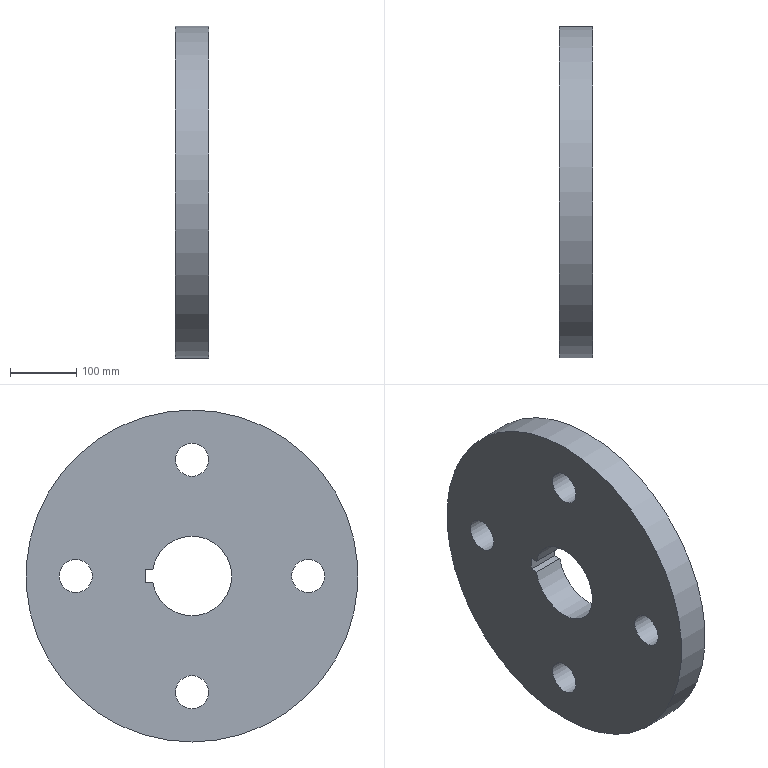Component | NX | ROTOR_DISC | 1 solid | 11 faces | box 50 x 500 x 500 mm | volume 8848841 mm3 | cylinder 6 | plane 5 | commonest cylinder face diameters 50 x4 500 x1 120 x1
STEP:
#1=CARTESIAN_POINT('',(0.,0.,0.));
#2=DIRECTION('',(0.,0.,1.));
#3=DIRECTION('',(1.,0.,0.));
#4=AXIS2_PLACEMENT_3D('',#1,#2,#3);
#5=CARTESIAN_POINT('',(641.458,-1109.721,829.997));
#6=VERTEX_POINT('',#5);
#7=CARTESIAN_POINT('',(641.458,-1098.711,829.997));
#8=VERTEX_POINT('',#7);
#9=CARTESIAN_POINT('',(641.458,-1109.721,829.997));
#10=DIRECTION('',(0.,1.,0.));
#11=VECTOR('',#10,1.);
#12=LINE('',#9,#11);
#13=CARTESIAN_POINT('',(591.458,-1109.721,829.997));
#14=DIRECTION('',(0.,0.,-1.));
#15=DIRECTION('',(-1.,0.,0.));
#16=AXIS2_PLACEMENT_3D('',#13,#14,#15);
#17=PLANE('',#16);
#18=CARTESIAN_POINT('',(-50.,0.));
#19=DIRECTION('',(0.,1.));
#20=VECTOR('',#19,1.);
#21=LINE('',#18,#20);
#22=(GEOMETRIC_REPRESENTATION_CONTEXT(2)PARAMETRIC_REPRESENTATION_CONTEXT()REPRESENTATION_CONTEXT('',''));
#23=DEFINITIONAL_REPRESENTATION('',(#21),#22);
#24=PCURVE('',#17,#23);
#25=CARTESIAN_POINT('',(641.458,-1168.882,839.997));
#26=DIRECTION('',(-1.,0.,0.));
#27=DIRECTION('',(0.,0.,1.));
#28=AXIS2_PLACEMENT_3D('',#25,#26,#27);
#29=PLANE('',#28);
#30=CARTESIAN_POINT('',(-10.,59.161));
#31=DIRECTION('',(0.,1.));
#32=VECTOR('',#31,1.);
#33=LINE('',#30,#32);
#34=(GEOMETRIC_REPRESENTATION_CONTEXT(2)PARAMETRIC_REPRESENTATION_CONTEXT()REPRESENTATION_CONTEXT('',''));
#35=DEFINITIONAL_REPRESENTATION('',(#33),#34);
#36=PCURVE('',#29,#35);
#37=SURFACE_CURVE('',#12,(#24,#36),.PCURVE_S1.);
#38=EDGE_CURVE('',#6,#8,#37,.T.);
#39=ORIENTED_EDGE('',*,*,#38,.T.);
#40=CARTESIAN_POINT('',(591.458,-1098.711,829.997));
#41=VERTEX_POINT('',#40);
#42=CARTESIAN_POINT('',(591.458,-1098.711,829.997));
#43=DIRECTION('',(1.,0.,0.));
#44=VECTOR('',#43,1.);
#45=LINE('',#42,#44);
#46=CARTESIAN_POINT('',(0.,11.01));
#47=DIRECTION('',(-1.,0.));
#48=VECTOR('',#47,1.);
#49=LINE('',#46,#48);
#50=(GEOMETRIC_REPRESENTATION_CONTEXT(2)PARAMETRIC_REPRESENTATION_CONTEXT()REPRESENTATION_CONTEXT('',''));
#51=DEFINITIONAL_REPRESENTATION('',(#49),#50);
#52=PCURVE('',#17,#51);
#53=CARTESIAN_POINT('',(591.458,-1098.711,829.997));
#54=DIRECTION('',(0.,1.,0.));
#55=DIRECTION('',(-1.,0.,0.));
#56=AXIS2_PLACEMENT_3D('',#53,#54,#55);
#57=PLANE('',#56);
#58=CARTESIAN_POINT('',(0.,0.));
#59=DIRECTION('',(-1.,0.));
#60=VECTOR('',#59,1.);
#61=LINE('',#58,#60);
#62=(GEOMETRIC_REPRESENTATION_CONTEXT(2)PARAMETRIC_REPRESENTATION_CONTEXT()REPRESENTATION_CONTEXT('',''));
#63=DEFINITIONAL_REPRESENTATION('',(#61),#62);
#64=PCURVE('',#57,#63);
#65=SURFACE_CURVE('',#45,(#52,#64),.PCURVE_S1.);
#66=EDGE_CURVE('',#41,#8,#65,.T.);
#67=ORIENTED_EDGE('',*,*,#66,.F.);
#68=CARTESIAN_POINT('',(591.458,-1109.721,829.997));
#69=VERTEX_POINT('',#68);
#70=CARTESIAN_POINT('',(591.458,-1109.721,829.997));
#71=DIRECTION('',(0.,1.,0.));
#72=VECTOR('',#71,1.);
#73=LINE('',#70,#72);
#74=CARTESIAN_POINT('',(0.,0.));
#75=DIRECTION('',(0.,1.));
#76=VECTOR('',#75,1.);
#77=LINE('',#74,#76);
#78=(GEOMETRIC_REPRESENTATION_CONTEXT(2)PARAMETRIC_REPRESENTATION_CONTEXT()REPRESENTATION_CONTEXT('',''));
#79=DEFINITIONAL_REPRESENTATION('',(#77),#78);
#80=PCURVE('',#17,#79);
#81=CARTESIAN_POINT('',(591.458,-1168.882,839.997));
#82=DIRECTION('',(-1.,0.,0.));
#83=DIRECTION('',(0.,0.,1.));
#84=AXIS2_PLACEMENT_3D('',#81,#82,#83);
#85=PLANE('',#84);
#86=CARTESIAN_POINT('',(-10.,59.161));
#87=DIRECTION('',(0.,1.));
#88=VECTOR('',#87,1.);
#89=LINE('',#86,#88);
#90=(GEOMETRIC_REPRESENTATION_CONTEXT(2)PARAMETRIC_REPRESENTATION_CONTEXT()REPRESENTATION_CONTEXT('',''));
#91=DEFINITIONAL_REPRESENTATION('',(#89),#90);
#92=PCURVE('',#85,#91);
#93=SURFACE_CURVE('',#73,(#80,#92),.PCURVE_S1.);
#94=EDGE_CURVE('',#69,#41,#93,.T.);
#95=ORIENTED_EDGE('',*,*,#94,.F.);
#96=CARTESIAN_POINT('',(591.458,-1109.721,829.997));
#97=DIRECTION('',(1.,0.,0.));
#98=VECTOR('',#97,1.);
#99=LINE('',#96,#98);
#100=CARTESIAN_POINT('',(0.,0.));
#101=DIRECTION('',(-1.,0.));
#102=VECTOR('',#101,1.);
#103=LINE('',#100,#102);
#104=(GEOMETRIC_REPRESENTATION_CONTEXT(2)PARAMETRIC_REPRESENTATION_CONTEXT()REPRESENTATION_CONTEXT('',''));
#105=DEFINITIONAL_REPRESENTATION('',(#103),#104);
#106=PCURVE('',#17,#105);
#107=CARTESIAN_POINT('',(591.458,-1168.882,839.997));
#108=DIRECTION('',(1.,0.,0.));
#109=DIRECTION('',(0.,0.,-1.));
#110=AXIS2_PLACEMENT_3D('',#107,#108,#109);
#111=CYLINDRICAL_SURFACE('',#110,60.);
#112=CARTESIAN_POINT('',(7.687,0.));
#113=DIRECTION('',(0.,1.));
#114=VECTOR('',#113,1.);
#115=LINE('',#112,#114);
#116=(GEOMETRIC_REPRESENTATION_CONTEXT(2)PARAMETRIC_REPRESENTATION_CONTEXT()REPRESENTATION_CONTEXT('',''));
#117=DEFINITIONAL_REPRESENTATION('',(#115),#116);
#118=PCURVE('',#111,#117);
#119=SURFACE_CURVE('',#99,(#106,#118),.PCURVE_S1.);
#120=EDGE_CURVE('',#69,#6,#119,.T.);
#121=ORIENTED_EDGE('',*,*,#120,.T.);
#122=EDGE_LOOP('',(#39,#67,#95,#121));
#123=FACE_BOUND('',#122,.T.);
#124=ADVANCED_FACE('',(#123),#17,.F.);
#125=CARTESIAN_POINT('',(641.458,-1098.711,849.997));
#126=VERTEX_POINT('',#125);
#127=CARTESIAN_POINT('',(641.458,-1098.711,829.997));
#128=DIRECTION('',(0.,0.,1.));
#129=VECTOR('',#128,1.);
#130=LINE('',#127,#129);
#131=CARTESIAN_POINT('',(-50.,0.));
#132=DIRECTION('',(0.,1.));
#133=VECTOR('',#132,1.);
#134=LINE('',#131,#133);
#135=(GEOMETRIC_REPRESENTATION_CONTEXT(2)PARAMETRIC_REPRESENTATION_CONTEXT()REPRESENTATION_CONTEXT('',''));
#136=DEFINITIONAL_REPRESENTATION('',(#134),#135);
#137=PCURVE('',#57,#136);
#138=CARTESIAN_POINT('',(-10.,70.171));
#139=DIRECTION('',(1.,0.));
#140=VECTOR('',#139,1.);
#141=LINE('',#138,#140);
#142=(GEOMETRIC_REPRESENTATION_CONTEXT(2)PARAMETRIC_REPRESENTATION_CONTEXT()REPRESENTATION_CONTEXT('',''));
#143=DEFINITIONAL_REPRESENTATION('',(#141),#142);
#144=PCURVE('',#29,#143);
#145=SURFACE_CURVE('',#130,(#137,#144),.PCURVE_S1.);
#146=EDGE_CURVE('',#8,#126,#145,.T.);
#147=ORIENTED_EDGE('',*,*,#146,.T.);
#148=CARTESIAN_POINT('',(591.458,-1098.711,849.997));
#149=VERTEX_POINT('',#148);
#150=CARTESIAN_POINT('',(591.458,-1098.711,849.997));
#151=DIRECTION('',(1.,0.,0.));
#152=VECTOR('',#151,1.);
#153=LINE('',#150,#152);
#154=CARTESIAN_POINT('',(0.,20.));
#155=DIRECTION('',(-1.,0.));
#156=VECTOR('',#155,1.);
#157=LINE('',#154,#156);
#158=(GEOMETRIC_REPRESENTATION_CONTEXT(2)PARAMETRIC_REPRESENTATION_CONTEXT()REPRESENTATION_CONTEXT('',''));
#159=DEFINITIONAL_REPRESENTATION('',(#157),#158);
#160=PCURVE('',#57,#159);
#161=CARTESIAN_POINT('',(591.458,-1098.711,849.997));
#162=DIRECTION('',(0.,0.,1.));
#163=DIRECTION('',(1.,0.,0.));
#164=AXIS2_PLACEMENT_3D('',#161,#162,#163);
#165=PLANE('',#164);
#166=CARTESIAN_POINT('',(0.,0.));
#167=DIRECTION('',(1.,0.));
#168=VECTOR('',#167,1.);
#169=LINE('',#166,#168);
#170=(GEOMETRIC_REPRESENTATION_CONTEXT(2)PARAMETRIC_REPRESENTATION_CONTEXT()REPRESENTATION_CONTEXT('',''));
#171=DEFINITIONAL_REPRESENTATION('',(#169),#170);
#172=PCURVE('',#165,#171);
#173=SURFACE_CURVE('',#153,(#160,#172),.PCURVE_S1.);
#174=EDGE_CURVE('',#149,#126,#173,.T.);
#175=ORIENTED_EDGE('',*,*,#174,.F.);
#176=CARTESIAN_POINT('',(591.458,-1098.711,829.997));
#177=DIRECTION('',(0.,0.,1.));
#178=VECTOR('',#177,1.);
#179=LINE('',#176,#178);
#180=CARTESIAN_POINT('',(0.,0.));
#181=DIRECTION('',(0.,1.));
#182=VECTOR('',#181,1.);
#183=LINE('',#180,#182);
#184=(GEOMETRIC_REPRESENTATION_CONTEXT(2)PARAMETRIC_REPRESENTATION_CONTEXT()REPRESENTATION_CONTEXT('',''));
#185=DEFINITIONAL_REPRESENTATION('',(#183),#184);
#186=PCURVE('',#57,#185);
#187=CARTESIAN_POINT('',(-10.,70.171));
#188=DIRECTION('',(1.,0.));
#189=VECTOR('',#188,1.);
#190=LINE('',#187,#189);
#191=(GEOMETRIC_REPRESENTATION_CONTEXT(2)PARAMETRIC_REPRESENTATION_CONTEXT()REPRESENTATION_CONTEXT('',''));
#192=DEFINITIONAL_REPRESENTATION('',(#190),#191);
#193=PCURVE('',#85,#192);
#194=SURFACE_CURVE('',#179,(#186,#193),.PCURVE_S1.);
#195=EDGE_CURVE('',#41,#149,#194,.T.);
#196=ORIENTED_EDGE('',*,*,#195,.F.);
#197=ORIENTED_EDGE('',*,*,#66,.T.);
#198=EDGE_LOOP('',(#147,#175,#196,#197));
#199=FACE_BOUND('',#198,.T.);
#200=ADVANCED_FACE('',(#199),#57,.F.);
#201=CARTESIAN_POINT('',(641.458,-1109.721,849.997));
#202=VERTEX_POINT('',#201);
#203=CARTESIAN_POINT('',(641.458,-1098.711,849.997));
#204=DIRECTION('',(0.,-1.,0.));
#205=VECTOR('',#204,1.);
#206=LINE('',#203,#205);
#207=CARTESIAN_POINT('',(50.,0.));
#208=DIRECTION('',(0.,-1.));
#209=VECTOR('',#208,1.);
#210=LINE('',#207,#209);
#211=(GEOMETRIC_REPRESENTATION_CONTEXT(2)PARAMETRIC_REPRESENTATION_CONTEXT()REPRESENTATION_CONTEXT('',''));
#212=DEFINITIONAL_REPRESENTATION('',(#210),#211);
#213=PCURVE('',#165,#212);
#214=CARTESIAN_POINT('',(10.,70.171));
#215=DIRECTION('',(0.,-1.));
#216=VECTOR('',#215,1.);
#217=LINE('',#214,#216);
#218=(GEOMETRIC_REPRESENTATION_CONTEXT(2)PARAMETRIC_REPRESENTATION_CONTEXT()REPRESENTATION_CONTEXT('',''));
#219=DEFINITIONAL_REPRESENTATION('',(#217),#218);
#220=PCURVE('',#29,#219);
#221=SURFACE_CURVE('',#206,(#213,#220),.PCURVE_S1.);
#222=EDGE_CURVE('',#126,#202,#221,.T.);
#223=ORIENTED_EDGE('',*,*,#222,.T.);
#224=CARTESIAN_POINT('',(591.458,-1109.721,849.997));
#225=VERTEX_POINT('',#224);
#226=CARTESIAN_POINT('',(591.458,-1109.721,849.997));
#227=DIRECTION('',(1.,0.,0.));
#228=VECTOR('',#227,1.);
#229=LINE('',#226,#228);
#230=CARTESIAN_POINT('',(0.,-11.01));
#231=DIRECTION('',(1.,0.));
#232=VECTOR('',#231,1.);
#233=LINE('',#230,#232);
#234=(GEOMETRIC_REPRESENTATION_CONTEXT(2)PARAMETRIC_REPRESENTATION_CONTEXT()REPRESENTATION_CONTEXT('',''));
#235=DEFINITIONAL_REPRESENTATION('',(#233),#234);
#236=PCURVE('',#165,#235);
#237=CARTESIAN_POINT('',(1.738,0.));
#238=DIRECTION('',(0.,1.));
#239=VECTOR('',#238,1.);
#240=LINE('',#237,#239);
#241=(GEOMETRIC_REPRESENTATION_CONTEXT(2)PARAMETRIC_REPRESENTATION_CONTEXT()REPRESENTATION_CONTEXT('',''));
#242=DEFINITIONAL_REPRESENTATION('',(#240),#241);
#243=PCURVE('',#111,#242);
#244=SURFACE_CURVE('',#229,(#236,#243),.PCURVE_S1.);
#245=EDGE_CURVE('',#225,#202,#244,.T.);
#246=ORIENTED_EDGE('',*,*,#245,.F.);
#247=CARTESIAN_POINT('',(591.458,-1098.711,849.997));
#248=DIRECTION('',(0.,-1.,0.));
#249=VECTOR('',#248,1.);
#250=LINE('',#247,#249);
#251=CARTESIAN_POINT('',(0.,0.));
#252=DIRECTION('',(0.,-1.));
#253=VECTOR('',#252,1.);
#254=LINE('',#251,#253);
#255=(GEOMETRIC_REPRESENTATION_CONTEXT(2)PARAMETRIC_REPRESENTATION_CONTEXT()REPRESENTATION_CONTEXT('',''));
#256=DEFINITIONAL_REPRESENTATION('',(#254),#255);
#257=PCURVE('',#165,#256);
#258=CARTESIAN_POINT('',(10.,70.171));
#259=DIRECTION('',(0.,-1.));
#260=VECTOR('',#259,1.);
#261=LINE('',#258,#260);
#262=(GEOMETRIC_REPRESENTATION_CONTEXT(2)PARAMETRIC_REPRESENTATION_CONTEXT()REPRESENTATION_CONTEXT('',''));
#263=DEFINITIONAL_REPRESENTATION('',(#261),#262);
#264=PCURVE('',#85,#263);
#265=SURFACE_CURVE('',#250,(#257,#264),.PCURVE_S1.);
#266=EDGE_CURVE('',#149,#225,#265,.T.);
#267=ORIENTED_EDGE('',*,*,#266,.F.);
#268=ORIENTED_EDGE('',*,*,#174,.T.);
#269=EDGE_LOOP('',(#223,#246,#267,#268));
#270=FACE_BOUND('',#269,.T.);
#271=ADVANCED_FACE('',(#270),#165,.F.);
#272=CARTESIAN_POINT('',(591.458,-1168.882,639.997));
#273=VERTEX_POINT('',#272);
#274=CARTESIAN_POINT('',(591.458,-1168.882,664.997));
#275=DIRECTION('',(-1.,0.,0.));
#276=DIRECTION('',(0.,0.,-1.));
#277=AXIS2_PLACEMENT_3D('',#274,#275,#276);
#278=CIRCLE('',#277,25.);
#279=CARTESIAN_POINT('',(591.458,-1168.882,664.997));
#280=DIRECTION('',(1.,0.,0.));
#281=DIRECTION('',(0.,0.,-1.));
#282=AXIS2_PLACEMENT_3D('',#279,#280,#281);
#283=CYLINDRICAL_SURFACE('',#282,25.);
#284=CARTESIAN_POINT('',(6.283,0.));
#285=DIRECTION('',(-1.,0.));
#286=VECTOR('',#285,1.);
#287=LINE('',#284,#286);
#288=(GEOMETRIC_REPRESENTATION_CONTEXT(2)PARAMETRIC_REPRESENTATION_CONTEXT()REPRESENTATION_CONTEXT('',''));
#289=DEFINITIONAL_REPRESENTATION('',(#287),#288);
#290=PCURVE('',#283,#289);
#291=CARTESIAN_POINT('',(-175.,0.));
#292=DIRECTION('',(-1.,0.));
#293=AXIS2_PLACEMENT_2D('',#291,#292);
#294=CIRCLE('',#293,25.);
#295=(GEOMETRIC_REPRESENTATION_CONTEXT(2)PARAMETRIC_REPRESENTATION_CONTEXT()REPRESENTATION_CONTEXT('',''));
#296=DEFINITIONAL_REPRESENTATION('',(#294),#295);
#297=PCURVE('',#85,#296);
#298=SURFACE_CURVE('',#278,(#290,#297),.PCURVE_S1.);
#299=EDGE_CURVE('',#273,#273,#298,.T.);
#300=ORIENTED_EDGE('',*,*,#299,.F.);
#301=CARTESIAN_POINT('',(641.458,-1168.882,639.997));
#302=VERTEX_POINT('',#301);
#303=CARTESIAN_POINT('',(591.458,-1168.882,639.997));
#304=CARTESIAN_POINT('',(641.458,-1168.882,639.997));
#305=B_SPLINE_CURVE_WITH_KNOTS('',1,(#303,#304),.UNSPECIFIED.,.F.,.F.,(2,2),(0.,50.),.PIECEWISE_BEZIER_KNOTS.);
#306=CARTESIAN_POINT('',(6.283,0.));
#307=DIRECTION('',(0.,1.));
#308=VECTOR('',#307,1.);
#309=LINE('',#306,#308);
#310=(GEOMETRIC_REPRESENTATION_CONTEXT(2)PARAMETRIC_REPRESENTATION_CONTEXT()REPRESENTATION_CONTEXT('',''));
#311=DEFINITIONAL_REPRESENTATION('',(#309),#310);
#312=PCURVE('',#283,#311);
#313=CARTESIAN_POINT('',(0.,0.));
#314=DIRECTION('',(0.,1.));
#315=VECTOR('',#314,1.);
#316=LINE('',#313,#315);
#317=(GEOMETRIC_REPRESENTATION_CONTEXT(2)PARAMETRIC_REPRESENTATION_CONTEXT()REPRESENTATION_CONTEXT('',''));
#318=DEFINITIONAL_REPRESENTATION('',(#316),#317);
#319=PCURVE('',#283,#318);
#320=SEAM_CURVE('',#305,(#312,#319),.PCURVE_S1.);
#321=EDGE_CURVE('',#273,#302,#320,.T.);
#322=ORIENTED_EDGE('',*,*,#321,.T.);
#323=CARTESIAN_POINT('',(641.458,-1168.882,664.997));
#324=DIRECTION('',(-1.,0.,0.));
#325=DIRECTION('',(0.,0.,-1.));
#326=AXIS2_PLACEMENT_3D('',#323,#324,#325);
#327=CIRCLE('',#326,25.);
#328=CARTESIAN_POINT('',(6.283,50.));
#329=DIRECTION('',(-1.,0.));
#330=VECTOR('',#329,1.);
#331=LINE('',#328,#330);
#332=(GEOMETRIC_REPRESENTATION_CONTEXT(2)PARAMETRIC_REPRESENTATION_CONTEXT()REPRESENTATION_CONTEXT('',''));
#333=DEFINITIONAL_REPRESENTATION('',(#331),#332);
#334=PCURVE('',#283,#333);
#335=CARTESIAN_POINT('',(-175.,0.));
#336=DIRECTION('',(-1.,0.));
#337=AXIS2_PLACEMENT_2D('',#335,#336);
#338=CIRCLE('',#337,25.);
#339=(GEOMETRIC_REPRESENTATION_CONTEXT(2)PARAMETRIC_REPRESENTATION_CONTEXT()REPRESENTATION_CONTEXT('',''));
#340=DEFINITIONAL_REPRESENTATION('',(#338),#339);
#341=PCURVE('',#29,#340);
#342=SURFACE_CURVE('',#327,(#334,#341),.PCURVE_S1.);
#343=EDGE_CURVE('',#302,#302,#342,.T.);
#344=ORIENTED_EDGE('',*,*,#343,.T.);
#345=ORIENTED_EDGE('',*,*,#321,.F.);
#346=EDGE_LOOP('',(#300,#322,#344,#345));
#347=FACE_BOUND('',#346,.F.);
#348=ADVANCED_FACE('',(#347),#283,.F.);
#349=CARTESIAN_POINT('',(591.458,-1368.882,839.997));
#350=VERTEX_POINT('',#349);
#351=CARTESIAN_POINT('',(591.458,-1343.882,839.997));
#352=DIRECTION('',(-1.,0.,0.));
#353=DIRECTION('',(0.,-1.,0.));
#354=AXIS2_PLACEMENT_3D('',#351,#352,#353);
#355=CIRCLE('',#354,25.);
#356=CARTESIAN_POINT('',(591.458,-1343.882,839.997));
#357=DIRECTION('',(1.,0.,0.));
#358=DIRECTION('',(0.,0.,-1.));
#359=AXIS2_PLACEMENT_3D('',#356,#357,#358);
#360=CYLINDRICAL_SURFACE('',#359,25.);
#361=CARTESIAN_POINT('',(10.996,0.));
#362=DIRECTION('',(-1.,0.));
#363=VECTOR('',#362,1.);
#364=LINE('',#361,#363);
#365=(GEOMETRIC_REPRESENTATION_CONTEXT(2)PARAMETRIC_REPRESENTATION_CONTEXT()REPRESENTATION_CONTEXT('',''));
#366=DEFINITIONAL_REPRESENTATION('',(#364),#365);
#367=PCURVE('',#360,#366);
#368=CARTESIAN_POINT('',(0.,-175.));
#369=DIRECTION('',(0.,-1.));
#370=AXIS2_PLACEMENT_2D('',#368,#369);
#371=CIRCLE('',#370,25.);
#372=(GEOMETRIC_REPRESENTATION_CONTEXT(2)PARAMETRIC_REPRESENTATION_CONTEXT()REPRESENTATION_CONTEXT('',''));
#373=DEFINITIONAL_REPRESENTATION('',(#371),#372);
#374=PCURVE('',#85,#373);
#375=SURFACE_CURVE('',#355,(#367,#374),.PCURVE_S1.);
#376=EDGE_CURVE('',#350,#350,#375,.T.);
#377=ORIENTED_EDGE('',*,*,#376,.F.);
#378=CARTESIAN_POINT('',(641.458,-1368.882,839.997));
#379=VERTEX_POINT('',#378);
#380=CARTESIAN_POINT('',(591.458,-1368.882,839.997));
#381=CARTESIAN_POINT('',(641.458,-1368.882,839.997));
#382=B_SPLINE_CURVE_WITH_KNOTS('',1,(#380,#381),.UNSPECIFIED.,.F.,.F.,(2,2),(0.,50.),.PIECEWISE_BEZIER_KNOTS.);
#383=CARTESIAN_POINT('',(10.996,0.));
#384=DIRECTION('',(0.,1.));
#385=VECTOR('',#384,1.);
#386=LINE('',#383,#385);
#387=(GEOMETRIC_REPRESENTATION_CONTEXT(2)PARAMETRIC_REPRESENTATION_CONTEXT()REPRESENTATION_CONTEXT('',''));
#388=DEFINITIONAL_REPRESENTATION('',(#386),#387);
#389=PCURVE('',#360,#388);
#390=CARTESIAN_POINT('',(4.712,0.));
#391=DIRECTION('',(0.,1.));
#392=VECTOR('',#391,1.);
#393=LINE('',#390,#392);
#394=(GEOMETRIC_REPRESENTATION_CONTEXT(2)PARAMETRIC_REPRESENTATION_CONTEXT()REPRESENTATION_CONTEXT('',''));
#395=DEFINITIONAL_REPRESENTATION('',(#393),#394);
#396=PCURVE('',#360,#395);
#397=SEAM_CURVE('',#382,(#389,#396),.PCURVE_S1.);
#398=EDGE_CURVE('',#350,#379,#397,.T.);
#399=ORIENTED_EDGE('',*,*,#398,.T.);
#400=CARTESIAN_POINT('',(641.458,-1343.882,839.997));
#401=DIRECTION('',(-1.,0.,0.));
#402=DIRECTION('',(0.,-1.,0.));
#403=AXIS2_PLACEMENT_3D('',#400,#401,#402);
#404=CIRCLE('',#403,25.);
#405=CARTESIAN_POINT('',(10.996,50.));
#406=DIRECTION('',(-1.,0.));
#407=VECTOR('',#406,1.);
#408=LINE('',#405,#407);
#409=(GEOMETRIC_REPRESENTATION_CONTEXT(2)PARAMETRIC_REPRESENTATION_CONTEXT()REPRESENTATION_CONTEXT('',''));
#410=DEFINITIONAL_REPRESENTATION('',(#408),#409);
#411=PCURVE('',#360,#410);
#412=CARTESIAN_POINT('',(0.,-175.));
#413=DIRECTION('',(0.,-1.));
#414=AXIS2_PLACEMENT_2D('',#412,#413);
#415=CIRCLE('',#414,25.);
#416=(GEOMETRIC_REPRESENTATION_CONTEXT(2)PARAMETRIC_REPRESENTATION_CONTEXT()REPRESENTATION_CONTEXT('',''));
#417=DEFINITIONAL_REPRESENTATION('',(#415),#416);
#418=PCURVE('',#29,#417);
#419=SURFACE_CURVE('',#404,(#411,#418),.PCURVE_S1.);
#420=EDGE_CURVE('',#379,#379,#419,.T.);
#421=ORIENTED_EDGE('',*,*,#420,.T.);
#422=ORIENTED_EDGE('',*,*,#398,.F.);
#423=EDGE_LOOP('',(#377,#399,#421,#422));
#424=FACE_BOUND('',#423,.F.);
#425=ADVANCED_FACE('',(#424),#360,.F.);
#426=CARTESIAN_POINT('',(591.458,-968.882,839.997));
#427=VERTEX_POINT('',#426);
#428=CARTESIAN_POINT('',(591.458,-993.882,839.997));
#429=DIRECTION('',(-1.,0.,0.));
#430=DIRECTION('',(0.,1.,0.));
#431=AXIS2_PLACEMENT_3D('',#428,#429,#430);
#432=CIRCLE('',#431,25.);
#433=CARTESIAN_POINT('',(591.458,-993.882,839.997));
#434=DIRECTION('',(1.,0.,0.));
#435=DIRECTION('',(0.,0.,-1.));
#436=AXIS2_PLACEMENT_3D('',#433,#434,#435);
#437=CYLINDRICAL_SURFACE('',#436,25.);
#438=CARTESIAN_POINT('',(7.854,0.));
#439=DIRECTION('',(-1.,0.));
#440=VECTOR('',#439,1.);
#441=LINE('',#438,#440);
#442=(GEOMETRIC_REPRESENTATION_CONTEXT(2)PARAMETRIC_REPRESENTATION_CONTEXT()REPRESENTATION_CONTEXT('',''));
#443=DEFINITIONAL_REPRESENTATION('',(#441),#442);
#444=PCURVE('',#437,#443);
#445=CARTESIAN_POINT('',(0.,175.));
#446=DIRECTION('',(0.,1.));
#447=AXIS2_PLACEMENT_2D('',#445,#446);
#448=CIRCLE('',#447,25.);
#449=(GEOMETRIC_REPRESENTATION_CONTEXT(2)PARAMETRIC_REPRESENTATION_CONTEXT()REPRESENTATION_CONTEXT('',''));
#450=DEFINITIONAL_REPRESENTATION('',(#448),#449);
#451=PCURVE('',#85,#450);
#452=SURFACE_CURVE('',#432,(#444,#451),.PCURVE_S1.);
#453=EDGE_CURVE('',#427,#427,#452,.T.);
#454=ORIENTED_EDGE('',*,*,#453,.F.);
#455=CARTESIAN_POINT('',(641.458,-968.882,839.997));
#456=VERTEX_POINT('',#455);
#457=CARTESIAN_POINT('',(591.458,-968.882,839.997));
#458=CARTESIAN_POINT('',(641.458,-968.882,839.997));
#459=B_SPLINE_CURVE_WITH_KNOTS('',1,(#457,#458),.UNSPECIFIED.,.F.,.F.,(2,2),(0.,50.),.PIECEWISE_BEZIER_KNOTS.);
#460=CARTESIAN_POINT('',(7.854,0.));
#461=DIRECTION('',(0.,1.));
#462=VECTOR('',#461,1.);
#463=LINE('',#460,#462);
#464=(GEOMETRIC_REPRESENTATION_CONTEXT(2)PARAMETRIC_REPRESENTATION_CONTEXT()REPRESENTATION_CONTEXT('',''));
#465=DEFINITIONAL_REPRESENTATION('',(#463),#464);
#466=PCURVE('',#437,#465);
#467=CARTESIAN_POINT('',(1.571,0.));
#468=DIRECTION('',(0.,1.));
#469=VECTOR('',#468,1.);
#470=LINE('',#467,#469);
#471=(GEOMETRIC_REPRESENTATION_CONTEXT(2)PARAMETRIC_REPRESENTATION_CONTEXT()REPRESENTATION_CONTEXT('',''));
#472=DEFINITIONAL_REPRESENTATION('',(#470),#471);
#473=PCURVE('',#437,#472);
#474=SEAM_CURVE('',#459,(#466,#473),.PCURVE_S1.);
#475=EDGE_CURVE('',#427,#456,#474,.T.);
#476=ORIENTED_EDGE('',*,*,#475,.T.);
#477=CARTESIAN_POINT('',(641.458,-993.882,839.997));
#478=DIRECTION('',(-1.,0.,0.));
#479=DIRECTION('',(0.,1.,0.));
#480=AXIS2_PLACEMENT_3D('',#477,#478,#479);
#481=CIRCLE('',#480,25.);
#482=CARTESIAN_POINT('',(7.854,50.));
#483=DIRECTION('',(-1.,0.));
#484=VECTOR('',#483,1.);
#485=LINE('',#482,#484);
#486=(GEOMETRIC_REPRESENTATION_CONTEXT(2)PARAMETRIC_REPRESENTATION_CONTEXT()REPRESENTATION_CONTEXT('',''));
#487=DEFINITIONAL_REPRESENTATION('',(#485),#486);
#488=PCURVE('',#437,#487);
#489=CARTESIAN_POINT('',(0.,175.));
#490=DIRECTION('',(0.,1.));
#491=AXIS2_PLACEMENT_2D('',#489,#490);
#492=CIRCLE('',#491,25.);
#493=(GEOMETRIC_REPRESENTATION_CONTEXT(2)PARAMETRIC_REPRESENTATION_CONTEXT()REPRESENTATION_CONTEXT('',''));
#494=DEFINITIONAL_REPRESENTATION('',(#492),#493);
#495=PCURVE('',#29,#494);
#496=SURFACE_CURVE('',#481,(#488,#495),.PCURVE_S1.);
#497=EDGE_CURVE('',#456,#456,#496,.T.);
#498=ORIENTED_EDGE('',*,*,#497,.T.);
#499=ORIENTED_EDGE('',*,*,#475,.F.);
#500=EDGE_LOOP('',(#454,#476,#498,#499));
#501=FACE_BOUND('',#500,.F.);
#502=ADVANCED_FACE('',(#501),#437,.F.);
#503=CARTESIAN_POINT('',(591.458,-1168.882,1039.997));
#504=VERTEX_POINT('',#503);
#505=CARTESIAN_POINT('',(591.458,-1168.882,1014.997));
#506=DIRECTION('',(-1.,0.,0.));
#507=DIRECTION('',(0.,0.,1.));
#508=AXIS2_PLACEMENT_3D('',#505,#506,#507);
#509=CIRCLE('',#508,25.);
#510=CARTESIAN_POINT('',(591.458,-1168.882,1014.997));
#511=DIRECTION('',(1.,0.,0.));
#512=DIRECTION('',(0.,0.,-1.));
#513=AXIS2_PLACEMENT_3D('',#510,#511,#512);
#514=CYLINDRICAL_SURFACE('',#513,25.);
#515=CARTESIAN_POINT('',(9.425,0.));
#516=DIRECTION('',(-1.,0.));
#517=VECTOR('',#516,1.);
#518=LINE('',#515,#517);
#519=(GEOMETRIC_REPRESENTATION_CONTEXT(2)PARAMETRIC_REPRESENTATION_CONTEXT()REPRESENTATION_CONTEXT('',''));
#520=DEFINITIONAL_REPRESENTATION('',(#518),#519);
#521=PCURVE('',#514,#520);
#522=CARTESIAN_POINT('',(175.,0.));
#523=DIRECTION('',(1.,0.));
#524=AXIS2_PLACEMENT_2D('',#522,#523);
#525=CIRCLE('',#524,25.);
#526=(GEOMETRIC_REPRESENTATION_CONTEXT(2)PARAMETRIC_REPRESENTATION_CONTEXT()REPRESENTATION_CONTEXT('',''));
#527=DEFINITIONAL_REPRESENTATION('',(#525),#526);
#528=PCURVE('',#85,#527);
#529=SURFACE_CURVE('',#509,(#521,#528),.PCURVE_S1.);
#530=EDGE_CURVE('',#504,#504,#529,.T.);
#531=ORIENTED_EDGE('',*,*,#530,.F.);
#532=CARTESIAN_POINT('',(641.458,-1168.882,1039.997));
#533=VERTEX_POINT('',#532);
#534=CARTESIAN_POINT('',(591.458,-1168.882,1039.997));
#535=CARTESIAN_POINT('',(641.458,-1168.882,1039.997));
#536=B_SPLINE_CURVE_WITH_KNOTS('',1,(#534,#535),.UNSPECIFIED.,.F.,.F.,(2,2),(0.,50.),.PIECEWISE_BEZIER_KNOTS.);
#537=CARTESIAN_POINT('',(9.425,0.));
#538=DIRECTION('',(0.,1.));
#539=VECTOR('',#538,1.);
#540=LINE('',#537,#539);
#541=(GEOMETRIC_REPRESENTATION_CONTEXT(2)PARAMETRIC_REPRESENTATION_CONTEXT()REPRESENTATION_CONTEXT('',''));
#542=DEFINITIONAL_REPRESENTATION('',(#540),#541);
#543=PCURVE('',#514,#542);
#544=CARTESIAN_POINT('',(3.142,0.));
#545=DIRECTION('',(0.,1.));
#546=VECTOR('',#545,1.);
#547=LINE('',#544,#546);
#548=(GEOMETRIC_REPRESENTATION_CONTEXT(2)PARAMETRIC_REPRESENTATION_CONTEXT()REPRESENTATION_CONTEXT('',''));
#549=DEFINITIONAL_REPRESENTATION('',(#547),#548);
#550=PCURVE('',#514,#549);
#551=SEAM_CURVE('',#536,(#543,#550),.PCURVE_S1.);
#552=EDGE_CURVE('',#504,#533,#551,.T.);
#553=ORIENTED_EDGE('',*,*,#552,.T.);
#554=CARTESIAN_POINT('',(641.458,-1168.882,1014.997));
#555=DIRECTION('',(-1.,0.,0.));
#556=DIRECTION('',(0.,0.,1.));
#557=AXIS2_PLACEMENT_3D('',#554,#555,#556);
#558=CIRCLE('',#557,25.);
#559=CARTESIAN_POINT('',(9.425,50.));
#560=DIRECTION('',(-1.,0.));
#561=VECTOR('',#560,1.);
#562=LINE('',#559,#561);
#563=(GEOMETRIC_REPRESENTATION_CONTEXT(2)PARAMETRIC_REPRESENTATION_CONTEXT()REPRESENTATION_CONTEXT('',''));
#564=DEFINITIONAL_REPRESENTATION('',(#562),#563);
#565=PCURVE('',#514,#564);
#566=CARTESIAN_POINT('',(175.,0.));
#567=DIRECTION('',(1.,0.));
#568=AXIS2_PLACEMENT_2D('',#566,#567);
#569=CIRCLE('',#568,25.);
#570=(GEOMETRIC_REPRESENTATION_CONTEXT(2)PARAMETRIC_REPRESENTATION_CONTEXT()REPRESENTATION_CONTEXT('',''));
#571=DEFINITIONAL_REPRESENTATION('',(#569),#570);
#572=PCURVE('',#29,#571);
#573=SURFACE_CURVE('',#558,(#565,#572),.PCURVE_S1.);
#574=EDGE_CURVE('',#533,#533,#573,.T.);
#575=ORIENTED_EDGE('',*,*,#574,.T.);
#576=ORIENTED_EDGE('',*,*,#552,.F.);
#577=EDGE_LOOP('',(#531,#553,#575,#576));
#578=FACE_BOUND('',#577,.F.);
#579=ADVANCED_FACE('',(#578),#514,.F.);
#580=CARTESIAN_POINT('',(591.458,-1168.882,1089.997));
#581=VERTEX_POINT('',#580);
#582=CARTESIAN_POINT('',(591.458,-1168.882,839.997));
#583=DIRECTION('',(-1.,0.,0.));
#584=DIRECTION('',(0.,0.,1.));
#585=AXIS2_PLACEMENT_3D('',#582,#583,#584);
#586=CIRCLE('',#585,250.);
#587=CARTESIAN_POINT('',(591.458,-1168.882,839.997));
#588=DIRECTION('',(1.,0.,0.));
#589=DIRECTION('',(0.,0.,-1.));
#590=AXIS2_PLACEMENT_3D('',#587,#588,#589);
#591=CYLINDRICAL_SURFACE('',#590,250.);
#592=CARTESIAN_POINT('',(9.425,0.));
#593=DIRECTION('',(-1.,0.));
#594=VECTOR('',#593,1.);
#595=LINE('',#592,#594);
#596=(GEOMETRIC_REPRESENTATION_CONTEXT(2)PARAMETRIC_REPRESENTATION_CONTEXT()REPRESENTATION_CONTEXT('',''));
#597=DEFINITIONAL_REPRESENTATION('',(#595),#596);
#598=PCURVE('',#591,#597);
#599=CARTESIAN_POINT('',(0.,0.));
#600=DIRECTION('',(1.,0.));
#601=AXIS2_PLACEMENT_2D('',#599,#600);
#602=CIRCLE('',#601,250.);
#603=(GEOMETRIC_REPRESENTATION_CONTEXT(2)PARAMETRIC_REPRESENTATION_CONTEXT()REPRESENTATION_CONTEXT('',''));
#604=DEFINITIONAL_REPRESENTATION('',(#602),#603);
#605=PCURVE('',#85,#604);
#606=SURFACE_CURVE('',#586,(#598,#605),.PCURVE_S1.);
#607=EDGE_CURVE('',#581,#581,#606,.T.);
#608=ORIENTED_EDGE('',*,*,#607,.F.);
#609=CARTESIAN_POINT('',(641.458,-1168.882,1089.997));
#610=VERTEX_POINT('',#609);
#611=CARTESIAN_POINT('',(591.458,-1168.882,1089.997));
#612=CARTESIAN_POINT('',(641.458,-1168.882,1089.997));
#613=B_SPLINE_CURVE_WITH_KNOTS('',1,(#611,#612),.UNSPECIFIED.,.F.,.F.,(2,2),(0.,50.),.PIECEWISE_BEZIER_KNOTS.);
#614=CARTESIAN_POINT('',(9.425,0.));
#615=DIRECTION('',(0.,1.));
#616=VECTOR('',#615,1.);
#617=LINE('',#614,#616);
#618=(GEOMETRIC_REPRESENTATION_CONTEXT(2)PARAMETRIC_REPRESENTATION_CONTEXT()REPRESENTATION_CONTEXT('',''));
#619=DEFINITIONAL_REPRESENTATION('',(#617),#618);
#620=PCURVE('',#591,#619);
#621=CARTESIAN_POINT('',(3.142,0.));
#622=DIRECTION('',(0.,1.));
#623=VECTOR('',#622,1.);
#624=LINE('',#621,#623);
#625=(GEOMETRIC_REPRESENTATION_CONTEXT(2)PARAMETRIC_REPRESENTATION_CONTEXT()REPRESENTATION_CONTEXT('',''));
#626=DEFINITIONAL_REPRESENTATION('',(#624),#625);
#627=PCURVE('',#591,#626);
#628=SEAM_CURVE('',#613,(#620,#627),.PCURVE_S1.);
#629=EDGE_CURVE('',#581,#610,#628,.T.);
#630=ORIENTED_EDGE('',*,*,#629,.T.);
#631=CARTESIAN_POINT('',(641.458,-1168.882,839.997));
#632=DIRECTION('',(-1.,0.,0.));
#633=DIRECTION('',(0.,0.,1.));
#634=AXIS2_PLACEMENT_3D('',#631,#632,#633);
#635=CIRCLE('',#634,250.);
#636=CARTESIAN_POINT('',(9.425,50.));
#637=DIRECTION('',(-1.,0.));
#638=VECTOR('',#637,1.);
#639=LINE('',#636,#638);
#640=(GEOMETRIC_REPRESENTATION_CONTEXT(2)PARAMETRIC_REPRESENTATION_CONTEXT()REPRESENTATION_CONTEXT('',''));
#641=DEFINITIONAL_REPRESENTATION('',(#639),#640);
#642=PCURVE('',#591,#641);
#643=CARTESIAN_POINT('',(0.,0.));
#644=DIRECTION('',(1.,0.));
#645=AXIS2_PLACEMENT_2D('',#643,#644);
#646=CIRCLE('',#645,250.);
#647=(GEOMETRIC_REPRESENTATION_CONTEXT(2)PARAMETRIC_REPRESENTATION_CONTEXT()REPRESENTATION_CONTEXT('',''));
#648=DEFINITIONAL_REPRESENTATION('',(#646),#647);
#649=PCURVE('',#29,#648);
#650=SURFACE_CURVE('',#635,(#642,#649),.PCURVE_S1.);
#651=EDGE_CURVE('',#610,#610,#650,.T.);
#652=ORIENTED_EDGE('',*,*,#651,.T.);
#653=ORIENTED_EDGE('',*,*,#629,.F.);
#654=EDGE_LOOP('',(#608,#630,#652,#653));
#655=FACE_BOUND('',#654,.T.);
#656=ADVANCED_FACE('',(#655),#591,.T.);
#657=ORIENTED_EDGE('',*,*,#245,.F.);
#658=CARTESIAN_POINT('',(591.458,-1168.882,839.997));
#659=DIRECTION('',(1.,0.,0.));
#660=DIRECTION('',(0.,0.,1.));
#661=AXIS2_PLACEMENT_3D('',#658,#659,#660);
#662=CIRCLE('',#661,60.);
#663=CARTESIAN_POINT('',(-3.142,0.));
#664=DIRECTION('',(1.,0.));
#665=VECTOR('',#664,1.);
#666=LINE('',#663,#665);
#667=(GEOMETRIC_REPRESENTATION_CONTEXT(2)PARAMETRIC_REPRESENTATION_CONTEXT()REPRESENTATION_CONTEXT('',''));
#668=DEFINITIONAL_REPRESENTATION('',(#666),#667);
#669=PCURVE('',#111,#668);
#670=CARTESIAN_POINT('',(60.,0.));
#671=CARTESIAN_POINT('',(60.,-103.923));
#672=CARTESIAN_POINT('',(-30.,-51.962));
#673=CARTESIAN_POINT('',(-120.,-0.));
#674=CARTESIAN_POINT('',(-30.,51.962));
#675=CARTESIAN_POINT('',(60.,103.923));
#676=CARTESIAN_POINT('',(60.,0.));
#677=(BOUNDED_CURVE()B_SPLINE_CURVE(2,(#670,#671,#672,#673,#674,#675,#676),.UNSPECIFIED.,.T.,.F.)B_SPLINE_CURVE_WITH_KNOTS((1,2,2,2,2,1),(-2.094,0.,2.094,4.189,6.283,8.378),.UNSPECIFIED.)CURVE()GEOMETRIC_REPRESENTATION_ITEM()RATIONAL_B_SPLINE_CURVE((1.,0.5,1.,0.5,1.,0.5,1.))REPRESENTATION_ITEM(''));
#678=(GEOMETRIC_REPRESENTATION_CONTEXT(2)PARAMETRIC_REPRESENTATION_CONTEXT()REPRESENTATION_CONTEXT('',''));
#679=DEFINITIONAL_REPRESENTATION('',(#677),#678);
#680=PCURVE('',#85,#679);
#681=SURFACE_CURVE('',#662,(#669,#680),.PCURVE_S1.);
#682=EDGE_CURVE('',#225,#69,#681,.T.);
#683=ORIENTED_EDGE('',*,*,#682,.T.);
#684=ORIENTED_EDGE('',*,*,#120,.T.);
#685=CARTESIAN_POINT('',(641.458,-1168.882,839.997));
#686=DIRECTION('',(1.,0.,0.));
#687=DIRECTION('',(0.,0.,1.));
#688=AXIS2_PLACEMENT_3D('',#685,#686,#687);
#689=CIRCLE('',#688,60.);
#690=CARTESIAN_POINT('',(-3.142,50.));
#691=DIRECTION('',(1.,0.));
#692=VECTOR('',#691,1.);
#693=LINE('',#690,#692);
#694=(GEOMETRIC_REPRESENTATION_CONTEXT(2)PARAMETRIC_REPRESENTATION_CONTEXT()REPRESENTATION_CONTEXT('',''));
#695=DEFINITIONAL_REPRESENTATION('',(#693),#694);
#696=PCURVE('',#111,#695);
#697=CARTESIAN_POINT('',(60.,0.));
#698=CARTESIAN_POINT('',(60.,-103.923));
#699=CARTESIAN_POINT('',(-30.,-51.962));
#700=CARTESIAN_POINT('',(-120.,-0.));
#701=CARTESIAN_POINT('',(-30.,51.962));
#702=CARTESIAN_POINT('',(60.,103.923));
#703=CARTESIAN_POINT('',(60.,0.));
#704=(BOUNDED_CURVE()B_SPLINE_CURVE(2,(#697,#698,#699,#700,#701,#702,#703),.UNSPECIFIED.,.T.,.F.)B_SPLINE_CURVE_WITH_KNOTS((1,2,2,2,2,1),(-2.094,0.,2.094,4.189,6.283,8.378),.UNSPECIFIED.)CURVE()GEOMETRIC_REPRESENTATION_ITEM()RATIONAL_B_SPLINE_CURVE((1.,0.5,1.,0.5,1.,0.5,1.))REPRESENTATION_ITEM(''));
#705=(GEOMETRIC_REPRESENTATION_CONTEXT(2)PARAMETRIC_REPRESENTATION_CONTEXT()REPRESENTATION_CONTEXT('',''));
#706=DEFINITIONAL_REPRESENTATION('',(#704),#705);
#707=PCURVE('',#29,#706);
#708=SURFACE_CURVE('',#689,(#696,#707),.PCURVE_S1.);
#709=EDGE_CURVE('',#202,#6,#708,.T.);
#710=ORIENTED_EDGE('',*,*,#709,.F.);
#711=EDGE_LOOP('',(#657,#683,#684,#710));
#712=FACE_BOUND('',#711,.F.);
#713=ADVANCED_FACE('',(#712),#111,.F.);
#714=ORIENTED_EDGE('',*,*,#607,.T.);
#715=EDGE_LOOP('',(#714));
#716=FACE_BOUND('',#715,.T.);
#717=ORIENTED_EDGE('',*,*,#530,.F.);
#718=EDGE_LOOP('',(#717));
#719=FACE_BOUND('',#718,.T.);
#720=ORIENTED_EDGE('',*,*,#453,.F.);
#721=EDGE_LOOP('',(#720));
#722=FACE_BOUND('',#721,.T.);
#723=ORIENTED_EDGE('',*,*,#376,.F.);
#724=EDGE_LOOP('',(#723));
#725=FACE_BOUND('',#724,.T.);
#726=ORIENTED_EDGE('',*,*,#299,.F.);
#727=EDGE_LOOP('',(#726));
#728=FACE_BOUND('',#727,.T.);
#729=ORIENTED_EDGE('',*,*,#94,.T.);
#730=ORIENTED_EDGE('',*,*,#195,.T.);
#731=ORIENTED_EDGE('',*,*,#266,.T.);
#732=ORIENTED_EDGE('',*,*,#682,.T.);
#733=EDGE_LOOP('',(#729,#730,#731,#732));
#734=FACE_BOUND('',#733,.T.);
#735=ADVANCED_FACE('',(#716,#719,#722,#725,#728,#734),#85,.T.);
#736=ORIENTED_EDGE('',*,*,#651,.F.);
#737=EDGE_LOOP('',(#736));
#738=FACE_BOUND('',#737,.T.);
#739=ORIENTED_EDGE('',*,*,#574,.T.);
#740=EDGE_LOOP('',(#739));
#741=FACE_BOUND('',#740,.T.);
#742=ORIENTED_EDGE('',*,*,#497,.T.);
#743=EDGE_LOOP('',(#742));
#744=FACE_BOUND('',#743,.T.);
#745=ORIENTED_EDGE('',*,*,#420,.T.);
#746=EDGE_LOOP('',(#745));
#747=FACE_BOUND('',#746,.T.);
#748=ORIENTED_EDGE('',*,*,#343,.T.);
#749=EDGE_LOOP('',(#748));
#750=FACE_BOUND('',#749,.T.);
#751=ORIENTED_EDGE('',*,*,#38,.F.);
#752=ORIENTED_EDGE('',*,*,#709,.F.);
#753=ORIENTED_EDGE('',*,*,#222,.F.);
#754=ORIENTED_EDGE('',*,*,#146,.F.);
#755=EDGE_LOOP('',(#751,#752,#753,#754));
#756=FACE_BOUND('',#755,.T.);
#757=ADVANCED_FACE('',(#738,#741,#744,#747,#750,#756),#29,.F.);
#758=CLOSED_SHELL('',(#124,#200,#271,#348,#425,#502,#579,#656,#713,#735,#757));
#759=MANIFOLD_SOLID_BREP('',#758);
#760=(LENGTH_UNIT()NAMED_UNIT(*)SI_UNIT(.MILLI.,.METRE.));
#761=UNCERTAINTY_MEASURE_WITH_UNIT(LENGTH_MEASURE(0.000005),#760,'','');
#762=(NAMED_UNIT(*)PLANE_ANGLE_UNIT()SI_UNIT($,.RADIAN.));
#763=(NAMED_UNIT(*)SI_UNIT($,.STERADIAN.)SOLID_ANGLE_UNIT());
#764=(GEOMETRIC_REPRESENTATION_CONTEXT(3)GLOBAL_UNCERTAINTY_ASSIGNED_CONTEXT((#761))GLOBAL_UNIT_ASSIGNED_CONTEXT((#760,#762,#763))REPRESENTATION_CONTEXT('',''));
#765=ADVANCED_BREP_SHAPE_REPRESENTATION('',(#4,#759),#764);